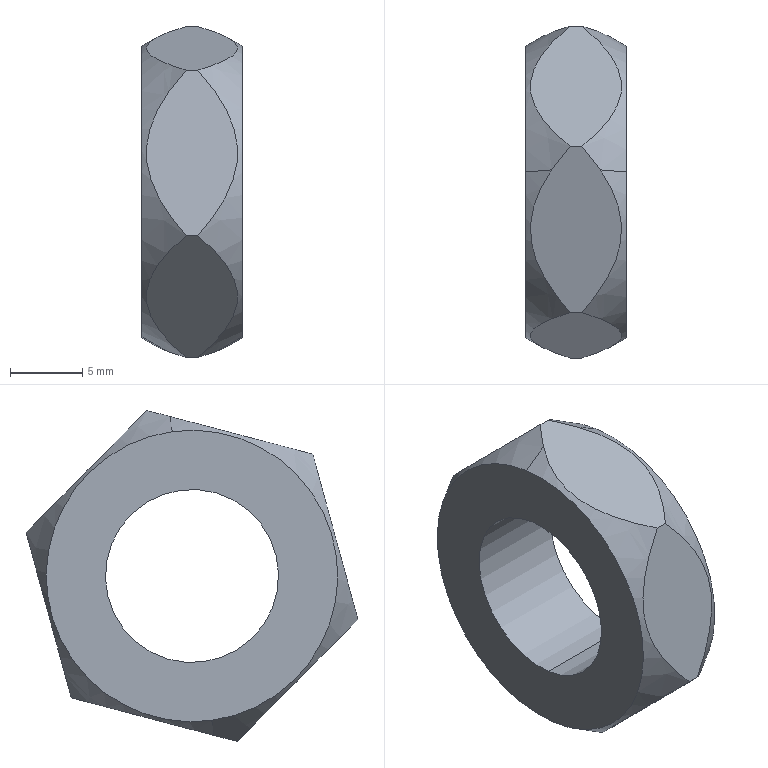Component | SolidWorks | NutM12-1 | 1 solid | 14 faces | box 7 x 23.01 x 22.95 mm | volume 1697 mm3 | plane 8 | cone 4 | cylinder 2 | commonest cylinder face diameters 12 x2
STEP:
#1=CARTESIAN_POINT('',(5.947,5.852,-0.9847));
#2=VERTEX_POINT('',#1);
#3=CARTESIAN_POINT('',(5.947,5.96,-0.1964));
#4=VERTEX_POINT('',#3);
#5=CARTESIAN_POINT('',(5.947,5.906,-0.5906));
#6=DIRECTION('',(1.,0.,0.));
#7=DIRECTION('',(0.,-0.1358,-0.9907));
#8=AXIS2_PLACEMENT_3D('',#5,#6,#7);
#9=CIRCLE('',#8,0.3978);
#10=EDGE_CURVE('',#2,#4,#9,.T.);
#11=ORIENTED_EDGE('',*,*,#10,.T.);
#12=CARTESIAN_POINT('',(6.018,5.965,-0.1556));
#13=VERTEX_POINT('',#12);
#14=CARTESIAN_POINT('',(5.947,5.96,-0.1964));
#15=DIRECTION('',(0.866,0.06788,0.4954));
#16=VECTOR('',#15,39.37);
#17=LINE('',#14,#16);
#18=EDGE_CURVE('',#4,#13,#17,.T.);
#19=ORIENTED_EDGE('',*,*,#18,.T.);
#20=CARTESIAN_POINT('',(6.069,6.029,-0.1388));
#21=VERTEX_POINT('',#20);
#22=CARTESIAN_POINT('',(6.069,6.029,-0.1388));
#23=CARTESIAN_POINT('',(6.051,6.008,-0.1442));
#24=CARTESIAN_POINT('',(6.034,5.987,-0.1497));
#25=CARTESIAN_POINT('',(6.018,5.965,-0.1556));
#26=B_SPLINE_CURVE_WITH_KNOTS('',3,(#22,#23,#24,#25),.UNSPECIFIED.,.F.,.F.,(4,4),(0.00000028,0.002105),.UNSPECIFIED.);
#27=EDGE_CURVE('',#21,#13,#26,.T.);
#28=ORIENTED_EDGE('',*,*,#27,.F.);
#29=CARTESIAN_POINT('',(6.069,6.358,-0.4715));
#30=VERTEX_POINT('',#29);
#31=CARTESIAN_POINT('',(6.069,6.358,-0.4715));
#32=CARTESIAN_POINT('',(6.054,6.347,-0.4597));
#33=CARTESIAN_POINT('',(6.041,6.335,-0.4475));
#34=CARTESIAN_POINT('',(6.015,6.31,-0.4222));
#35=CARTESIAN_POINT('',(6.004,6.297,-0.4091));
#36=CARTESIAN_POINT('',(5.984,6.269,-0.3814));
#37=CARTESIAN_POINT('',(5.975,6.255,-0.3667));
#38=CARTESIAN_POINT('',(5.966,6.232,-0.3442));
#39=CARTESIAN_POINT('',(5.964,6.225,-0.3366));
#40=CARTESIAN_POINT('',(5.961,6.209,-0.3211));
#41=CARTESIAN_POINT('',(5.96,6.202,-0.3131));
#42=CARTESIAN_POINT('',(5.96,6.178,-0.2897));
#43=CARTESIAN_POINT('',(5.963,6.163,-0.2743));
#44=CARTESIAN_POINT('',(5.975,6.133,-0.2439));
#45=CARTESIAN_POINT('',(5.983,6.119,-0.2295));
#46=CARTESIAN_POINT('',(6.003,6.091,-0.2018));
#47=CARTESIAN_POINT('',(6.015,6.078,-0.1885));
#48=CARTESIAN_POINT('',(6.041,6.053,-0.1629));
#49=CARTESIAN_POINT('',(6.054,6.041,-0.1507));
#50=CARTESIAN_POINT('',(6.069,6.029,-0.1388));
#51=B_SPLINE_CURVE_WITH_KNOTS('',3,(#31,#32,#33,#34,#35,#36,#37,#38,#39,#40,#41,#42,#43,#44,#45,#46,#47,#48,#49,#50),.UNSPECIFIED.,.F.,.F.,(4,2,2,2,2,2,2,2,2,4),(0.00000033,0.001663,0.003326,0.004989,0.005821,0.006652,0.008315,0.009978,0.01164,0.0133),.UNSPECIFIED.);
#52=EDGE_CURVE('',#30,#21,#51,.T.);
#53=ORIENTED_EDGE('',*,*,#52,.F.);
#54=CARTESIAN_POINT('',(6.069,6.235,-0.9232));
#55=VERTEX_POINT('',#54);
#56=CARTESIAN_POINT('',(6.069,6.235,-0.9232));
#57=CARTESIAN_POINT('',(6.054,6.239,-0.9072));
#58=CARTESIAN_POINT('',(6.041,6.244,-0.8907));
#59=CARTESIAN_POINT('',(6.015,6.253,-0.8563));
#60=CARTESIAN_POINT('',(6.004,6.258,-0.8385));
#61=CARTESIAN_POINT('',(5.984,6.268,-0.8009));
#62=CARTESIAN_POINT('',(5.975,6.274,-0.7809));
#63=CARTESIAN_POINT('',(5.966,6.282,-0.7504));
#64=CARTESIAN_POINT('',(5.964,6.285,-0.74));
#65=CARTESIAN_POINT('',(5.961,6.291,-0.7189));
#66=CARTESIAN_POINT('',(5.96,6.294,-0.7082));
#67=CARTESIAN_POINT('',(5.96,6.302,-0.6763));
#68=CARTESIAN_POINT('',(5.963,6.308,-0.6554));
#69=CARTESIAN_POINT('',(5.975,6.319,-0.6142));
#70=CARTESIAN_POINT('',(5.983,6.325,-0.5946));
#71=CARTESIAN_POINT('',(6.003,6.335,-0.557));
#72=CARTESIAN_POINT('',(6.015,6.34,-0.5389));
#73=CARTESIAN_POINT('',(6.041,6.349,-0.5042));
#74=CARTESIAN_POINT('',(6.054,6.354,-0.4876));
#75=CARTESIAN_POINT('',(6.069,6.358,-0.4715));
#76=B_SPLINE_CURVE_WITH_KNOTS('',3,(#56,#57,#58,#59,#60,#61,#62,#63,#64,#65,#66,#67,#68,#69,#70,#71,#72,#73,#74,#75),.UNSPECIFIED.,.F.,.F.,(4,2,2,2,2,2,2,2,2,4),(0.00000026,0.001663,0.003326,0.004989,0.00582,0.006652,0.008315,0.009978,0.01164,0.0133),.UNSPECIFIED.);
#77=EDGE_CURVE('',#55,#30,#76,.T.);
#78=ORIENTED_EDGE('',*,*,#77,.F.);
#79=CARTESIAN_POINT('',(6.018,5.846,-1.026));
#80=VERTEX_POINT('',#79);
#81=CARTESIAN_POINT('',(6.018,5.846,-1.026));
#82=CARTESIAN_POINT('',(6.008,5.861,-1.022));
#83=CARTESIAN_POINT('',(5.999,5.876,-1.018));
#84=CARTESIAN_POINT('',(5.982,5.908,-1.009));
#85=CARTESIAN_POINT('',(5.975,5.925,-1.005));
#86=CARTESIAN_POINT('',(5.968,5.951,-0.998));
#87=CARTESIAN_POINT('',(5.966,5.959,-0.9957));
#88=CARTESIAN_POINT('',(5.962,5.977,-0.991));
#89=CARTESIAN_POINT('',(5.961,5.986,-0.9887));
#90=CARTESIAN_POINT('',(5.96,6.013,-0.9816));
#91=CARTESIAN_POINT('',(5.961,6.031,-0.9769));
#92=CARTESIAN_POINT('',(5.967,6.066,-0.9677));
#93=CARTESIAN_POINT('',(5.972,6.084,-0.9631));
#94=CARTESIAN_POINT('',(5.986,6.117,-0.9543));
#95=CARTESIAN_POINT('',(5.994,6.133,-0.9501));
#96=CARTESIAN_POINT('',(6.013,6.164,-0.942));
#97=CARTESIAN_POINT('',(6.023,6.179,-0.9381));
#98=CARTESIAN_POINT('',(6.045,6.208,-0.9305));
#99=CARTESIAN_POINT('',(6.057,6.221,-0.9268));
#100=CARTESIAN_POINT('',(6.069,6.235,-0.9232));
#101=B_SPLINE_CURVE_WITH_KNOTS('',3,(#81,#82,#83,#84,#85,#86,#87,#88,#89,#90,#91,#92,#93,#94,#95,#96,#97,#98,#99,#100),.UNSPECIFIED.,.F.,.F.,(4,2,2,2,2,2,2,2,2,4),(0.002105,0.003505,0.004905,0.005605,0.006304,0.007704,0.009104,0.0105,0.0119,0.0133),.UNSPECIFIED.);
#102=EDGE_CURVE('',#80,#55,#101,.T.);
#103=ORIENTED_EDGE('',*,*,#102,.F.);
#104=CARTESIAN_POINT('',(5.947,5.852,-0.9847));
#105=DIRECTION('',(0.866,-0.06788,-0.4954));
#106=VECTOR('',#105,39.37);
#107=LINE('',#104,#106);
#108=EDGE_CURVE('',#2,#80,#107,.T.);
#109=ORIENTED_EDGE('',*,*,#108,.F.);
#110=EDGE_LOOP('',(#11,#19,#28,#53,#78,#103,#109));
#111=FACE_OUTER_BOUND('',#110,.T.);
#112=CARTESIAN_POINT('',(5.947,5.906,-0.5906));
#113=DIRECTION('',(1.,0.,0.));
#114=DIRECTION('',(0.,-0.1358,-0.9907));
#115=AXIS2_PLACEMENT_3D('',#112,#113,#114);
#116=CONICAL_SURFACE('',#115,0.3978,0.5236);
#117=ADVANCED_FACE('',(#111),#116,.T.);
#118=CARTESIAN_POINT('',(6.223,5.96,-0.1964));
#119=VERTEX_POINT('',#118);
#120=CARTESIAN_POINT('',(6.223,5.852,-0.9847));
#121=VERTEX_POINT('',#120);
#122=CARTESIAN_POINT('',(6.223,5.906,-0.5906));
#123=DIRECTION('',(1.,0.,0.));
#124=DIRECTION('',(0.,-0.1358,-0.9907));
#125=AXIS2_PLACEMENT_3D('',#122,#123,#124);
#126=CIRCLE('',#125,0.3978);
#127=EDGE_CURVE('',#119,#121,#126,.T.);
#128=ORIENTED_EDGE('',*,*,#127,.F.);
#129=CARTESIAN_POINT('',(6.151,5.965,-0.1556));
#130=VERTEX_POINT('',#129);
#131=CARTESIAN_POINT('',(6.223,5.96,-0.1964));
#132=DIRECTION('',(-0.866,0.06788,0.4954));
#133=VECTOR('',#132,39.37);
#134=LINE('',#131,#133);
#135=EDGE_CURVE('',#119,#130,#134,.T.);
#136=ORIENTED_EDGE('',*,*,#135,.T.);
#137=CARTESIAN_POINT('',(6.101,5.576,-0.2579));
#138=VERTEX_POINT('',#137);
#139=CARTESIAN_POINT('',(6.151,5.965,-0.1556));
#140=CARTESIAN_POINT('',(6.161,5.95,-0.1595));
#141=CARTESIAN_POINT('',(6.171,5.935,-0.1635));
#142=CARTESIAN_POINT('',(6.187,5.903,-0.1719));
#143=CARTESIAN_POINT('',(6.194,5.886,-0.1764));
#144=CARTESIAN_POINT('',(6.202,5.86,-0.1831));
#145=CARTESIAN_POINT('',(6.204,5.852,-0.1854));
#146=CARTESIAN_POINT('',(6.207,5.834,-0.1901));
#147=CARTESIAN_POINT('',(6.208,5.825,-0.1924));
#148=CARTESIAN_POINT('',(6.21,5.798,-0.1995));
#149=CARTESIAN_POINT('',(6.209,5.78,-0.2042));
#150=CARTESIAN_POINT('',(6.202,5.745,-0.2134));
#151=CARTESIAN_POINT('',(6.197,5.728,-0.218));
#152=CARTESIAN_POINT('',(6.184,5.694,-0.2268));
#153=CARTESIAN_POINT('',(6.175,5.678,-0.231));
#154=CARTESIAN_POINT('',(6.157,5.647,-0.2391));
#155=CARTESIAN_POINT('',(6.146,5.632,-0.243));
#156=CARTESIAN_POINT('',(6.124,5.604,-0.2506));
#157=CARTESIAN_POINT('',(6.113,5.59,-0.2543));
#158=CARTESIAN_POINT('',(6.101,5.576,-0.2579));
#159=B_SPLINE_CURVE_WITH_KNOTS('',3,(#139,#140,#141,#142,#143,#144,#145,#146,#147,#148,#149,#150,#151,#152,#153,#154,#155,#156,#157,#158),.UNSPECIFIED.,.F.,.F.,(4,2,2,2,2,2,2,2,2,4),(0.002105,0.003505,0.004905,0.005605,0.006304,0.007704,0.009104,0.0105,0.0119,0.0133),.UNSPECIFIED.);
#160=EDGE_CURVE('',#130,#138,#159,.T.);
#161=ORIENTED_EDGE('',*,*,#160,.T.);
#162=CARTESIAN_POINT('',(6.101,5.453,-0.7096));
#163=VERTEX_POINT('',#162);
#164=CARTESIAN_POINT('',(6.101,5.576,-0.2579));
#165=CARTESIAN_POINT('',(6.115,5.572,-0.2739));
#166=CARTESIAN_POINT('',(6.129,5.567,-0.2905));
#167=CARTESIAN_POINT('',(6.154,5.558,-0.3248));
#168=CARTESIAN_POINT('',(6.166,5.553,-0.3426));
#169=CARTESIAN_POINT('',(6.186,5.543,-0.3802));
#170=CARTESIAN_POINT('',(6.194,5.537,-0.4002));
#171=CARTESIAN_POINT('',(6.203,5.529,-0.4307));
#172=CARTESIAN_POINT('',(6.205,5.526,-0.4411));
#173=CARTESIAN_POINT('',(6.208,5.52,-0.4622));
#174=CARTESIAN_POINT('',(6.209,5.517,-0.4729));
#175=CARTESIAN_POINT('',(6.209,5.509,-0.5048));
#176=CARTESIAN_POINT('',(6.206,5.503,-0.5257));
#177=CARTESIAN_POINT('',(6.194,5.492,-0.5669));
#178=CARTESIAN_POINT('',(6.186,5.486,-0.5866));
#179=CARTESIAN_POINT('',(6.166,5.476,-0.6241));
#180=CARTESIAN_POINT('',(6.154,5.471,-0.6422));
#181=CARTESIAN_POINT('',(6.129,5.462,-0.6769));
#182=CARTESIAN_POINT('',(6.115,5.457,-0.6935));
#183=CARTESIAN_POINT('',(6.101,5.453,-0.7096));
#184=B_SPLINE_CURVE_WITH_KNOTS('',3,(#164,#165,#166,#167,#168,#169,#170,#171,#172,#173,#174,#175,#176,#177,#178,#179,#180,#181,#182,#183),.UNSPECIFIED.,.F.,.F.,(4,2,2,2,2,2,2,2,2,4),(0.00000026,0.001663,0.003326,0.004989,0.00582,0.006652,0.008315,0.009978,0.01164,0.0133),.UNSPECIFIED.);
#185=EDGE_CURVE('',#138,#163,#184,.T.);
#186=ORIENTED_EDGE('',*,*,#185,.T.);
#187=CARTESIAN_POINT('',(6.101,5.782,-1.042));
#188=VERTEX_POINT('',#187);
#189=CARTESIAN_POINT('',(6.101,5.453,-0.7096));
#190=CARTESIAN_POINT('',(6.115,5.464,-0.7214));
#191=CARTESIAN_POINT('',(6.129,5.476,-0.7336));
#192=CARTESIAN_POINT('',(6.154,5.501,-0.7589));
#193=CARTESIAN_POINT('',(6.166,5.514,-0.772));
#194=CARTESIAN_POINT('',(6.186,5.542,-0.7997));
#195=CARTESIAN_POINT('',(6.194,5.556,-0.8144));
#196=CARTESIAN_POINT('',(6.203,5.579,-0.8369));
#197=CARTESIAN_POINT('',(6.205,5.586,-0.8445));
#198=CARTESIAN_POINT('',(6.208,5.602,-0.8601));
#199=CARTESIAN_POINT('',(6.209,5.61,-0.868));
#200=CARTESIAN_POINT('',(6.209,5.633,-0.8914));
#201=CARTESIAN_POINT('',(6.206,5.648,-0.9068));
#202=CARTESIAN_POINT('',(6.194,5.678,-0.9372));
#203=CARTESIAN_POINT('',(6.186,5.692,-0.9517));
#204=CARTESIAN_POINT('',(6.166,5.72,-0.9793));
#205=CARTESIAN_POINT('',(6.154,5.733,-0.9926));
#206=CARTESIAN_POINT('',(6.129,5.758,-1.018));
#207=CARTESIAN_POINT('',(6.115,5.77,-1.03));
#208=CARTESIAN_POINT('',(6.101,5.782,-1.042));
#209=B_SPLINE_CURVE_WITH_KNOTS('',3,(#189,#190,#191,#192,#193,#194,#195,#196,#197,#198,#199,#200,#201,#202,#203,#204,#205,#206,#207,#208),.UNSPECIFIED.,.F.,.F.,(4,2,2,2,2,2,2,2,2,4),(0.00000033,0.001663,0.003326,0.004989,0.005821,0.006652,0.008315,0.009978,0.01164,0.0133),.UNSPECIFIED.);
#210=EDGE_CURVE('',#163,#188,#209,.T.);
#211=ORIENTED_EDGE('',*,*,#210,.T.);
#212=CARTESIAN_POINT('',(6.151,5.846,-1.026));
#213=VERTEX_POINT('',#212);
#214=CARTESIAN_POINT('',(6.101,5.782,-1.042));
#215=CARTESIAN_POINT('',(6.119,5.803,-1.037));
#216=CARTESIAN_POINT('',(6.136,5.824,-1.031));
#217=CARTESIAN_POINT('',(6.151,5.846,-1.026));
#218=B_SPLINE_CURVE_WITH_KNOTS('',3,(#214,#215,#216,#217),.UNSPECIFIED.,.F.,.F.,(4,4),(0.00000028,0.002105),.UNSPECIFIED.);
#219=EDGE_CURVE('',#188,#213,#218,.T.);
#220=ORIENTED_EDGE('',*,*,#219,.T.);
#221=CARTESIAN_POINT('',(6.223,5.852,-0.9847));
#222=DIRECTION('',(-0.866,-0.06788,-0.4954));
#223=VECTOR('',#222,39.37);
#224=LINE('',#221,#223);
#225=EDGE_CURVE('',#121,#213,#224,.T.);
#226=ORIENTED_EDGE('',*,*,#225,.F.);
#227=EDGE_LOOP('',(#128,#136,#161,#186,#211,#220,#226));
#228=FACE_OUTER_BOUND('',#227,.T.);
#229=CARTESIAN_POINT('',(6.223,5.906,-0.5906));
#230=DIRECTION('',(-1.,0.,0.));
#231=DIRECTION('',(0.,-0.1358,-0.9907));
#232=AXIS2_PLACEMENT_3D('',#229,#230,#231);
#233=CONICAL_SURFACE('',#232,0.3978,0.5236);
#234=ADVANCED_FACE('',(#228),#233,.T.);
#235=CARTESIAN_POINT('',(6.223,5.938,-0.3565));
#236=VERTEX_POINT('',#235);
#237=CARTESIAN_POINT('',(6.223,5.873,-0.8246));
#238=VERTEX_POINT('',#237);
#239=CARTESIAN_POINT('',(6.223,5.906,-0.5906));
#240=DIRECTION('',(1.,0.,0.));
#241=DIRECTION('',(0.,-0.1358,-0.9907));
#242=AXIS2_PLACEMENT_3D('',#239,#240,#241);
#243=CIRCLE('',#242,0.2362);
#244=EDGE_CURVE('',#236,#238,#243,.T.);
#245=ORIENTED_EDGE('',*,*,#244,.T.);
#246=CARTESIAN_POINT('',(5.947,5.873,-0.8246));
#247=VERTEX_POINT('',#246);
#248=CARTESIAN_POINT('',(6.223,5.873,-0.8246));
#249=DIRECTION('',(-1.,0.,0.));
#250=VECTOR('',#249,39.37);
#251=LINE('',#248,#250);
#252=EDGE_CURVE('',#238,#247,#251,.T.);
#253=ORIENTED_EDGE('',*,*,#252,.T.);
#254=CARTESIAN_POINT('',(5.947,5.938,-0.3565));
#255=VERTEX_POINT('',#254);
#256=CARTESIAN_POINT('',(5.947,5.906,-0.5906));
#257=DIRECTION('',(1.,0.,0.));
#258=DIRECTION('',(0.,-0.1358,-0.9907));
#259=AXIS2_PLACEMENT_3D('',#256,#257,#258);
#260=CIRCLE('',#259,0.2362);
#261=EDGE_CURVE('',#255,#247,#260,.T.);
#262=ORIENTED_EDGE('',*,*,#261,.F.);
#263=CARTESIAN_POINT('',(6.223,5.938,-0.3565));
#264=DIRECTION('',(-1.,0.,0.));
#265=VECTOR('',#264,39.37);
#266=LINE('',#263,#265);
#267=EDGE_CURVE('',#236,#255,#266,.T.);
#268=ORIENTED_EDGE('',*,*,#267,.F.);
#269=EDGE_LOOP('',(#245,#253,#262,#268));
#270=FACE_OUTER_BOUND('',#269,.T.);
#271=CARTESIAN_POINT('',(6.223,5.906,-0.5906));
#272=DIRECTION('',(-1.,0.,0.));
#273=DIRECTION('',(0.,0.1358,0.9907));
#274=AXIS2_PLACEMENT_3D('',#271,#272,#273);
#275=CYLINDRICAL_SURFACE('',#274,0.2362);
#276=ADVANCED_FACE('',(#270),#275,.F.);
#277=ORIENTED_EDGE('',*,*,#261,.T.);
#278=CARTESIAN_POINT('',(5.947,5.906,-0.5906));
#279=DIRECTION('',(1.,0.,0.));
#280=DIRECTION('',(0.,-0.1358,-0.9907));
#281=AXIS2_PLACEMENT_3D('',#278,#279,#280);
#282=CIRCLE('',#281,0.2362);
#283=EDGE_CURVE('',#247,#255,#282,.T.);
#284=ORIENTED_EDGE('',*,*,#283,.T.);
#285=EDGE_LOOP('',(#277,#284));
#286=FACE_BOUND('',#285,.T.);
#287=ORIENTED_EDGE('',*,*,#10,.F.);
#288=CARTESIAN_POINT('',(5.947,5.906,-0.5906));
#289=DIRECTION('',(1.,0.,0.));
#290=DIRECTION('',(0.,-0.1358,-0.9907));
#291=AXIS2_PLACEMENT_3D('',#288,#289,#290);
#292=CIRCLE('',#291,0.3978);
#293=EDGE_CURVE('',#4,#2,#292,.T.);
#294=ORIENTED_EDGE('',*,*,#293,.F.);
#295=EDGE_LOOP('',(#287,#294));
#296=FACE_OUTER_BOUND('',#295,.T.);
#297=CARTESIAN_POINT('',(5.947,0.1348,0.7962));
#298=DIRECTION('',(1.,0.,0.));
#299=DIRECTION('',(0.,-0.1358,-0.9907));
#300=AXIS2_PLACEMENT_3D('',#297,#298,#299);
#301=PLANE('',#300);
#302=ADVANCED_FACE('',(#286,#296),#301,.F.);
#303=ORIENTED_EDGE('',*,*,#244,.F.);
#304=CARTESIAN_POINT('',(6.223,5.906,-0.5906));
#305=DIRECTION('',(1.,0.,0.));
#306=DIRECTION('',(0.,-0.1358,-0.9907));
#307=AXIS2_PLACEMENT_3D('',#304,#305,#306);
#308=CIRCLE('',#307,0.2362);
#309=EDGE_CURVE('',#238,#236,#308,.T.);
#310=ORIENTED_EDGE('',*,*,#309,.F.);
#311=EDGE_LOOP('',(#303,#310));
#312=FACE_BOUND('',#311,.T.);
#313=CARTESIAN_POINT('',(6.223,5.906,-0.5906));
#314=DIRECTION('',(1.,0.,0.));
#315=DIRECTION('',(0.,-0.1358,-0.9907));
#316=AXIS2_PLACEMENT_3D('',#313,#314,#315);
#317=CIRCLE('',#316,0.3978);
#318=EDGE_CURVE('',#121,#119,#317,.T.);
#319=ORIENTED_EDGE('',*,*,#318,.T.);
#320=ORIENTED_EDGE('',*,*,#127,.T.);
#321=EDGE_LOOP('',(#319,#320));
#322=FACE_OUTER_BOUND('',#321,.T.);
#323=CARTESIAN_POINT('',(6.223,0.1348,0.7962));
#324=DIRECTION('',(1.,0.,0.));
#325=DIRECTION('',(0.,-0.1358,-0.9907));
#326=AXIS2_PLACEMENT_3D('',#323,#324,#325);
#327=PLANE('',#326);
#328=ADVANCED_FACE('',(#312,#322),#327,.T.);
#329=CARTESIAN_POINT('',(6.069,5.782,-1.042));
#330=VERTEX_POINT('',#329);
#331=CARTESIAN_POINT('',(6.223,5.782,-1.042));
#332=DIRECTION('',(-1.,0.,0.));
#333=VECTOR('',#332,39.37);
#334=LINE('',#331,#333);
#335=EDGE_CURVE('',#188,#330,#334,.T.);
#336=ORIENTED_EDGE('',*,*,#335,.T.);
#337=CARTESIAN_POINT('',(6.069,5.782,-1.042));
#338=CARTESIAN_POINT('',(6.051,5.803,-1.037));
#339=CARTESIAN_POINT('',(6.034,5.824,-1.031));
#340=CARTESIAN_POINT('',(6.018,5.846,-1.026));
#341=B_SPLINE_CURVE_WITH_KNOTS('',3,(#337,#338,#339,#340),.UNSPECIFIED.,.F.,.F.,(4,4),(0.00000028,0.002105),.UNSPECIFIED.);
#342=EDGE_CURVE('',#330,#80,#341,.T.);
#343=ORIENTED_EDGE('',*,*,#342,.T.);
#344=ORIENTED_EDGE('',*,*,#102,.T.);
#345=CARTESIAN_POINT('',(6.101,6.235,-0.9232));
#346=VERTEX_POINT('',#345);
#347=CARTESIAN_POINT('',(6.223,6.235,-0.9232));
#348=DIRECTION('',(-1.,0.,0.));
#349=VECTOR('',#348,39.37);
#350=LINE('',#347,#349);
#351=EDGE_CURVE('',#346,#55,#350,.T.);
#352=ORIENTED_EDGE('',*,*,#351,.F.);
#353=CARTESIAN_POINT('',(6.151,5.846,-1.026));
#354=CARTESIAN_POINT('',(6.161,5.861,-1.022));
#355=CARTESIAN_POINT('',(6.171,5.876,-1.018));
#356=CARTESIAN_POINT('',(6.187,5.908,-1.009));
#357=CARTESIAN_POINT('',(6.194,5.925,-1.005));
#358=CARTESIAN_POINT('',(6.202,5.951,-0.998));
#359=CARTESIAN_POINT('',(6.204,5.959,-0.9957));
#360=CARTESIAN_POINT('',(6.207,5.977,-0.991));
#361=CARTESIAN_POINT('',(6.208,5.986,-0.9887));
#362=CARTESIAN_POINT('',(6.21,6.013,-0.9816));
#363=CARTESIAN_POINT('',(6.209,6.031,-0.9769));
#364=CARTESIAN_POINT('',(6.202,6.066,-0.9677));
#365=CARTESIAN_POINT('',(6.197,6.084,-0.9631));
#366=CARTESIAN_POINT('',(6.184,6.117,-0.9543));
#367=CARTESIAN_POINT('',(6.175,6.133,-0.9501));
#368=CARTESIAN_POINT('',(6.157,6.164,-0.942));
#369=CARTESIAN_POINT('',(6.146,6.179,-0.9381));
#370=CARTESIAN_POINT('',(6.124,6.208,-0.9305));
#371=CARTESIAN_POINT('',(6.113,6.221,-0.9268));
#372=CARTESIAN_POINT('',(6.101,6.235,-0.9232));
#373=B_SPLINE_CURVE_WITH_KNOTS('',3,(#353,#354,#355,#356,#357,#358,#359,#360,#361,#362,#363,#364,#365,#366,#367,#368,#369,#370,#371,#372),.UNSPECIFIED.,.F.,.F.,(4,2,2,2,2,2,2,2,2,4),(0.002105,0.003505,0.004905,0.005605,0.006304,0.007704,0.009104,0.0105,0.0119,0.0133),.UNSPECIFIED.);
#374=EDGE_CURVE('',#213,#346,#373,.T.);
#375=ORIENTED_EDGE('',*,*,#374,.F.);
#376=ORIENTED_EDGE('',*,*,#219,.F.);
#377=EDGE_LOOP('',(#336,#343,#344,#352,#375,#376));
#378=FACE_OUTER_BOUND('',#377,.T.);
#379=CARTESIAN_POINT('',(6.223,5.782,-1.042));
#380=DIRECTION('',(0.,-0.2543,0.9671));
#381=DIRECTION('',(0.,-0.9671,-0.2543));
#382=AXIS2_PLACEMENT_3D('',#379,#380,#381);
#383=PLANE('',#382);
#384=ADVANCED_FACE('',(#378),#383,.F.);
#385=ORIENTED_EDGE('',*,*,#351,.T.);
#386=ORIENTED_EDGE('',*,*,#77,.T.);
#387=CARTESIAN_POINT('',(6.101,6.358,-0.4715));
#388=VERTEX_POINT('',#387);
#389=CARTESIAN_POINT('',(6.223,6.358,-0.4715));
#390=DIRECTION('',(-1.,0.,0.));
#391=VECTOR('',#390,39.37);
#392=LINE('',#389,#391);
#393=EDGE_CURVE('',#388,#30,#392,.T.);
#394=ORIENTED_EDGE('',*,*,#393,.F.);
#395=CARTESIAN_POINT('',(6.101,6.235,-0.9232));
#396=CARTESIAN_POINT('',(6.115,6.239,-0.9072));
#397=CARTESIAN_POINT('',(6.129,6.244,-0.8907));
#398=CARTESIAN_POINT('',(6.154,6.253,-0.8563));
#399=CARTESIAN_POINT('',(6.166,6.258,-0.8385));
#400=CARTESIAN_POINT('',(6.186,6.268,-0.8009));
#401=CARTESIAN_POINT('',(6.194,6.274,-0.7809));
#402=CARTESIAN_POINT('',(6.203,6.282,-0.7504));
#403=CARTESIAN_POINT('',(6.205,6.285,-0.74));
#404=CARTESIAN_POINT('',(6.208,6.291,-0.7189));
#405=CARTESIAN_POINT('',(6.209,6.294,-0.7082));
#406=CARTESIAN_POINT('',(6.209,6.302,-0.6763));
#407=CARTESIAN_POINT('',(6.206,6.308,-0.6554));
#408=CARTESIAN_POINT('',(6.194,6.319,-0.6142));
#409=CARTESIAN_POINT('',(6.186,6.325,-0.5946));
#410=CARTESIAN_POINT('',(6.166,6.335,-0.557));
#411=CARTESIAN_POINT('',(6.154,6.34,-0.5389));
#412=CARTESIAN_POINT('',(6.129,6.349,-0.5042));
#413=CARTESIAN_POINT('',(6.115,6.354,-0.4876));
#414=CARTESIAN_POINT('',(6.101,6.358,-0.4715));
#415=B_SPLINE_CURVE_WITH_KNOTS('',3,(#395,#396,#397,#398,#399,#400,#401,#402,#403,#404,#405,#406,#407,#408,#409,#410,#411,#412,#413,#414),.UNSPECIFIED.,.F.,.F.,(4,2,2,2,2,2,2,2,2,4),(0.00000026,0.001663,0.003326,0.004989,0.00582,0.006652,0.008315,0.009978,0.01164,0.0133),.UNSPECIFIED.);
#416=EDGE_CURVE('',#346,#388,#415,.T.);
#417=ORIENTED_EDGE('',*,*,#416,.F.);
#418=EDGE_LOOP('',(#385,#386,#394,#417));
#419=FACE_OUTER_BOUND('',#418,.T.);
#420=CARTESIAN_POINT('',(6.223,6.235,-0.9232));
#421=DIRECTION('',(0.,-0.9647,0.2634));
#422=DIRECTION('',(0.,-0.2634,-0.9647));
#423=AXIS2_PLACEMENT_3D('',#420,#421,#422);
#424=PLANE('',#423);
#425=ADVANCED_FACE('',(#419),#424,.F.);
#426=ORIENTED_EDGE('',*,*,#393,.T.);
#427=ORIENTED_EDGE('',*,*,#52,.T.);
#428=CARTESIAN_POINT('',(6.101,6.029,-0.1388));
#429=VERTEX_POINT('',#428);
#430=CARTESIAN_POINT('',(6.223,6.029,-0.1388));
#431=DIRECTION('',(-1.,0.,0.));
#432=VECTOR('',#431,39.37);
#433=LINE('',#430,#432);
#434=EDGE_CURVE('',#429,#21,#433,.T.);
#435=ORIENTED_EDGE('',*,*,#434,.F.);
#436=CARTESIAN_POINT('',(6.101,6.358,-0.4715));
#437=CARTESIAN_POINT('',(6.115,6.347,-0.4597));
#438=CARTESIAN_POINT('',(6.129,6.335,-0.4475));
#439=CARTESIAN_POINT('',(6.154,6.31,-0.4222));
#440=CARTESIAN_POINT('',(6.166,6.297,-0.4091));
#441=CARTESIAN_POINT('',(6.186,6.269,-0.3814));
#442=CARTESIAN_POINT('',(6.194,6.255,-0.3667));
#443=CARTESIAN_POINT('',(6.203,6.232,-0.3442));
#444=CARTESIAN_POINT('',(6.205,6.225,-0.3366));
#445=CARTESIAN_POINT('',(6.208,6.209,-0.3211));
#446=CARTESIAN_POINT('',(6.209,6.202,-0.3131));
#447=CARTESIAN_POINT('',(6.209,6.178,-0.2897));
#448=CARTESIAN_POINT('',(6.206,6.163,-0.2743));
#449=CARTESIAN_POINT('',(6.194,6.133,-0.2439));
#450=CARTESIAN_POINT('',(6.186,6.119,-0.2295));
#451=CARTESIAN_POINT('',(6.166,6.091,-0.2018));
#452=CARTESIAN_POINT('',(6.154,6.078,-0.1885));
#453=CARTESIAN_POINT('',(6.129,6.053,-0.1629));
#454=CARTESIAN_POINT('',(6.115,6.041,-0.1507));
#455=CARTESIAN_POINT('',(6.101,6.029,-0.1388));
#456=B_SPLINE_CURVE_WITH_KNOTS('',3,(#436,#437,#438,#439,#440,#441,#442,#443,#444,#445,#446,#447,#448,#449,#450,#451,#452,#453,#454,#455),.UNSPECIFIED.,.F.,.F.,(4,2,2,2,2,2,2,2,2,4),(0.00000033,0.001663,0.003326,0.004989,0.005821,0.006652,0.008315,0.009978,0.01164,0.0133),.UNSPECIFIED.);
#457=EDGE_CURVE('',#388,#429,#456,.T.);
#458=ORIENTED_EDGE('',*,*,#457,.F.);
#459=EDGE_LOOP('',(#426,#427,#435,#458));
#460=FACE_OUTER_BOUND('',#459,.T.);
#461=CARTESIAN_POINT('',(6.223,6.358,-0.4715));
#462=DIRECTION('',(0.,-0.7104,-0.7038));
#463=DIRECTION('',(0.,0.7038,-0.7104));
#464=AXIS2_PLACEMENT_3D('',#461,#462,#463);
#465=PLANE('',#464);
#466=ADVANCED_FACE('',(#460),#465,.F.);
#467=ORIENTED_EDGE('',*,*,#434,.T.);
#468=ORIENTED_EDGE('',*,*,#27,.T.);
#469=CARTESIAN_POINT('',(6.069,5.576,-0.2579));
#470=VERTEX_POINT('',#469);
#471=CARTESIAN_POINT('',(6.018,5.965,-0.1556));
#472=CARTESIAN_POINT('',(6.008,5.95,-0.1595));
#473=CARTESIAN_POINT('',(5.999,5.935,-0.1635));
#474=CARTESIAN_POINT('',(5.982,5.903,-0.1719));
#475=CARTESIAN_POINT('',(5.975,5.886,-0.1764));
#476=CARTESIAN_POINT('',(5.968,5.86,-0.1831));
#477=CARTESIAN_POINT('',(5.966,5.852,-0.1854));
#478=CARTESIAN_POINT('',(5.962,5.834,-0.1901));
#479=CARTESIAN_POINT('',(5.961,5.825,-0.1924));
#480=CARTESIAN_POINT('',(5.96,5.798,-0.1995));
#481=CARTESIAN_POINT('',(5.961,5.78,-0.2042));
#482=CARTESIAN_POINT('',(5.967,5.745,-0.2134));
#483=CARTESIAN_POINT('',(5.972,5.728,-0.218));
#484=CARTESIAN_POINT('',(5.986,5.694,-0.2268));
#485=CARTESIAN_POINT('',(5.994,5.678,-0.231));
#486=CARTESIAN_POINT('',(6.013,5.647,-0.2391));
#487=CARTESIAN_POINT('',(6.023,5.632,-0.243));
#488=CARTESIAN_POINT('',(6.045,5.604,-0.2506));
#489=CARTESIAN_POINT('',(6.057,5.59,-0.2543));
#490=CARTESIAN_POINT('',(6.069,5.576,-0.2579));
#491=B_SPLINE_CURVE_WITH_KNOTS('',3,(#471,#472,#473,#474,#475,#476,#477,#478,#479,#480,#481,#482,#483,#484,#485,#486,#487,#488,#489,#490),.UNSPECIFIED.,.F.,.F.,(4,2,2,2,2,2,2,2,2,4),(0.002105,0.003505,0.004905,0.005605,0.006304,0.007704,0.009104,0.0105,0.0119,0.0133),.UNSPECIFIED.);
#492=EDGE_CURVE('',#13,#470,#491,.T.);
#493=ORIENTED_EDGE('',*,*,#492,.T.);
#494=CARTESIAN_POINT('',(6.223,5.576,-0.2579));
#495=DIRECTION('',(-1.,0.,0.));
#496=VECTOR('',#495,39.37);
#497=LINE('',#494,#496);
#498=EDGE_CURVE('',#138,#470,#497,.T.);
#499=ORIENTED_EDGE('',*,*,#498,.F.);
#500=ORIENTED_EDGE('',*,*,#160,.F.);
#501=CARTESIAN_POINT('',(6.101,6.029,-0.1388));
#502=CARTESIAN_POINT('',(6.119,6.008,-0.1442));
#503=CARTESIAN_POINT('',(6.136,5.987,-0.1497));
#504=CARTESIAN_POINT('',(6.151,5.965,-0.1556));
#505=B_SPLINE_CURVE_WITH_KNOTS('',3,(#501,#502,#503,#504),.UNSPECIFIED.,.F.,.F.,(4,4),(0.00000028,0.002105),.UNSPECIFIED.);
#506=EDGE_CURVE('',#429,#130,#505,.T.);
#507=ORIENTED_EDGE('',*,*,#506,.F.);
#508=EDGE_LOOP('',(#467,#468,#493,#499,#500,#507));
#509=FACE_OUTER_BOUND('',#508,.T.);
#510=CARTESIAN_POINT('',(6.223,6.029,-0.1388));
#511=DIRECTION('',(0.,0.2543,-0.9671));
#512=DIRECTION('',(0.,0.9671,0.2543));
#513=AXIS2_PLACEMENT_3D('',#510,#511,#512);
#514=PLANE('',#513);
#515=ADVANCED_FACE('',(#509),#514,.F.);
#516=ORIENTED_EDGE('',*,*,#498,.T.);
#517=CARTESIAN_POINT('',(6.069,5.453,-0.7096));
#518=VERTEX_POINT('',#517);
#519=CARTESIAN_POINT('',(6.069,5.576,-0.2579));
#520=CARTESIAN_POINT('',(6.054,5.572,-0.2739));
#521=CARTESIAN_POINT('',(6.041,5.567,-0.2905));
#522=CARTESIAN_POINT('',(6.015,5.558,-0.3248));
#523=CARTESIAN_POINT('',(6.004,5.553,-0.3426));
#524=CARTESIAN_POINT('',(5.984,5.543,-0.3802));
#525=CARTESIAN_POINT('',(5.975,5.537,-0.4002));
#526=CARTESIAN_POINT('',(5.966,5.529,-0.4307));
#527=CARTESIAN_POINT('',(5.964,5.526,-0.4411));
#528=CARTESIAN_POINT('',(5.961,5.52,-0.4622));
#529=CARTESIAN_POINT('',(5.96,5.517,-0.4729));
#530=CARTESIAN_POINT('',(5.96,5.509,-0.5048));
#531=CARTESIAN_POINT('',(5.963,5.503,-0.5257));
#532=CARTESIAN_POINT('',(5.975,5.492,-0.5669));
#533=CARTESIAN_POINT('',(5.983,5.486,-0.5866));
#534=CARTESIAN_POINT('',(6.003,5.476,-0.6241));
#535=CARTESIAN_POINT('',(6.015,5.471,-0.6422));
#536=CARTESIAN_POINT('',(6.041,5.462,-0.6769));
#537=CARTESIAN_POINT('',(6.054,5.457,-0.6935));
#538=CARTESIAN_POINT('',(6.069,5.453,-0.7096));
#539=B_SPLINE_CURVE_WITH_KNOTS('',3,(#519,#520,#521,#522,#523,#524,#525,#526,#527,#528,#529,#530,#531,#532,#533,#534,#535,#536,#537,#538),.UNSPECIFIED.,.F.,.F.,(4,2,2,2,2,2,2,2,2,4),(0.00000026,0.001663,0.003326,0.004989,0.00582,0.006652,0.008315,0.009978,0.01164,0.0133),.UNSPECIFIED.);
#540=EDGE_CURVE('',#470,#518,#539,.T.);
#541=ORIENTED_EDGE('',*,*,#540,.T.);
#542=CARTESIAN_POINT('',(6.223,5.453,-0.7096));
#543=DIRECTION('',(-1.,0.,0.));
#544=VECTOR('',#543,39.37);
#545=LINE('',#542,#544);
#546=EDGE_CURVE('',#163,#518,#545,.T.);
#547=ORIENTED_EDGE('',*,*,#546,.F.);
#548=ORIENTED_EDGE('',*,*,#185,.F.);
#549=EDGE_LOOP('',(#516,#541,#547,#548));
#550=FACE_OUTER_BOUND('',#549,.T.);
#551=CARTESIAN_POINT('',(6.223,5.576,-0.2579));
#552=DIRECTION('',(0.,0.9647,-0.2634));
#553=DIRECTION('',(0.,0.2634,0.9647));
#554=AXIS2_PLACEMENT_3D('',#551,#552,#553);
#555=PLANE('',#554);
#556=ADVANCED_FACE('',(#550),#555,.F.);
#557=ORIENTED_EDGE('',*,*,#546,.T.);
#558=CARTESIAN_POINT('',(6.069,5.453,-0.7096));
#559=CARTESIAN_POINT('',(6.054,5.464,-0.7214));
#560=CARTESIAN_POINT('',(6.041,5.476,-0.7336));
#561=CARTESIAN_POINT('',(6.015,5.501,-0.7589));
#562=CARTESIAN_POINT('',(6.004,5.514,-0.772));
#563=CARTESIAN_POINT('',(5.984,5.542,-0.7997));
#564=CARTESIAN_POINT('',(5.975,5.556,-0.8144));
#565=CARTESIAN_POINT('',(5.966,5.579,-0.8369));
#566=CARTESIAN_POINT('',(5.964,5.586,-0.8445));
#567=CARTESIAN_POINT('',(5.961,5.602,-0.8601));
#568=CARTESIAN_POINT('',(5.96,5.61,-0.868));
#569=CARTESIAN_POINT('',(5.96,5.633,-0.8914));
#570=CARTESIAN_POINT('',(5.963,5.648,-0.9068));
#571=CARTESIAN_POINT('',(5.975,5.678,-0.9372));
#572=CARTESIAN_POINT('',(5.983,5.692,-0.9517));
#573=CARTESIAN_POINT('',(6.003,5.72,-0.9793));
#574=CARTESIAN_POINT('',(6.015,5.733,-0.9926));
#575=CARTESIAN_POINT('',(6.041,5.758,-1.018));
#576=CARTESIAN_POINT('',(6.054,5.77,-1.03));
#577=CARTESIAN_POINT('',(6.069,5.782,-1.042));
#578=B_SPLINE_CURVE_WITH_KNOTS('',3,(#558,#559,#560,#561,#562,#563,#564,#565,#566,#567,#568,#569,#570,#571,#572,#573,#574,#575,#576,#577),.UNSPECIFIED.,.F.,.F.,(4,2,2,2,2,2,2,2,2,4),(0.00000033,0.001663,0.003326,0.004989,0.005821,0.006652,0.008315,0.009978,0.01164,0.0133),.UNSPECIFIED.);
#579=EDGE_CURVE('',#518,#330,#578,.T.);
#580=ORIENTED_EDGE('',*,*,#579,.T.);
#581=ORIENTED_EDGE('',*,*,#335,.F.);
#582=ORIENTED_EDGE('',*,*,#210,.F.);
#583=EDGE_LOOP('',(#557,#580,#581,#582));
#584=FACE_OUTER_BOUND('',#583,.T.);
#585=CARTESIAN_POINT('',(6.223,5.453,-0.7096));
#586=DIRECTION('',(0.,0.7104,0.7038));
#587=DIRECTION('',(0.,-0.7038,0.7104));
#588=AXIS2_PLACEMENT_3D('',#585,#586,#587);
#589=PLANE('',#588);
#590=ADVANCED_FACE('',(#584),#589,.F.);
#591=ORIENTED_EDGE('',*,*,#252,.F.);
#592=ORIENTED_EDGE('',*,*,#309,.T.);
#593=ORIENTED_EDGE('',*,*,#267,.T.);
#594=ORIENTED_EDGE('',*,*,#283,.F.);
#595=EDGE_LOOP('',(#591,#592,#593,#594));
#596=FACE_OUTER_BOUND('',#595,.T.);
#597=CARTESIAN_POINT('',(6.223,5.906,-0.5906));
#598=DIRECTION('',(-1.,0.,0.));
#599=DIRECTION('',(0.,0.1358,0.9907));
#600=AXIS2_PLACEMENT_3D('',#597,#598,#599);
#601=CYLINDRICAL_SURFACE('',#600,0.2362);
#602=ADVANCED_FACE('',(#596),#601,.F.);
#603=ORIENTED_EDGE('',*,*,#135,.F.);
#604=ORIENTED_EDGE('',*,*,#318,.F.);
#605=ORIENTED_EDGE('',*,*,#225,.T.);
#606=ORIENTED_EDGE('',*,*,#374,.T.);
#607=ORIENTED_EDGE('',*,*,#416,.T.);
#608=ORIENTED_EDGE('',*,*,#457,.T.);
#609=ORIENTED_EDGE('',*,*,#506,.T.);
#610=EDGE_LOOP('',(#603,#604,#605,#606,#607,#608,#609));
#611=FACE_OUTER_BOUND('',#610,.T.);
#612=CARTESIAN_POINT('',(6.223,5.906,-0.5906));
#613=DIRECTION('',(-1.,0.,0.));
#614=DIRECTION('',(0.,-0.1358,-0.9907));
#615=AXIS2_PLACEMENT_3D('',#612,#613,#614);
#616=CONICAL_SURFACE('',#615,0.3978,0.5236);
#617=ADVANCED_FACE('',(#611),#616,.T.);
#618=ORIENTED_EDGE('',*,*,#18,.F.);
#619=ORIENTED_EDGE('',*,*,#293,.T.);
#620=ORIENTED_EDGE('',*,*,#108,.T.);
#621=ORIENTED_EDGE('',*,*,#342,.F.);
#622=ORIENTED_EDGE('',*,*,#579,.F.);
#623=ORIENTED_EDGE('',*,*,#540,.F.);
#624=ORIENTED_EDGE('',*,*,#492,.F.);
#625=EDGE_LOOP('',(#618,#619,#620,#621,#622,#623,#624));
#626=FACE_OUTER_BOUND('',#625,.T.);
#627=CARTESIAN_POINT('',(5.947,5.906,-0.5906));
#628=DIRECTION('',(1.,0.,0.));
#629=DIRECTION('',(0.,-0.1358,-0.9907));
#630=AXIS2_PLACEMENT_3D('',#627,#628,#629);
#631=CONICAL_SURFACE('',#630,0.3978,0.5236);
#632=ADVANCED_FACE('',(#626),#631,.T.);
#633=CLOSED_SHELL('',(#117,#234,#276,#302,#328,#384,#425,#466,#515,#556,#590,#602,#617,#632));
#634=MANIFOLD_SOLID_BREP('',#633);
#635=CARTESIAN_POINT('',(0.,0.,0.));
#636=DIRECTION('',(0.,0.,1.));
#637=DIRECTION('',(1.,0.,0.));
#638=AXIS2_PLACEMENT_3D('',#635,#636,#637);
#639=(LENGTH_UNIT()NAMED_UNIT(*)SI_UNIT($,.METRE.));
#640=LENGTH_MEASURE_WITH_UNIT(LENGTH_MEASURE(0.0254),#639);
#641=DIMENSIONAL_EXPONENTS(1.,0.,0.,0.,0.,0.,0.);
#642=(CONVERSION_BASED_UNIT('',#640)LENGTH_UNIT()NAMED_UNIT(#641));
#643=UNCERTAINTY_MEASURE_WITH_UNIT(LENGTH_MEASURE(0.00001),#642,'','');
#644=(NAMED_UNIT(*)PLANE_ANGLE_UNIT()SI_UNIT($,.RADIAN.));
#645=(NAMED_UNIT(*)SI_UNIT($,.STERADIAN.)SOLID_ANGLE_UNIT());
#646=(GEOMETRIC_REPRESENTATION_CONTEXT(3)GLOBAL_UNCERTAINTY_ASSIGNED_CONTEXT((#643))GLOBAL_UNIT_ASSIGNED_CONTEXT((#642,#644,#645))REPRESENTATION_CONTEXT('',''));
#647=ADVANCED_BREP_SHAPE_REPRESENTATION('',(#634,#638),#646);
#648=COLOUR_RGB('',0.7922,0.8196,0.9333);
#649=FILL_AREA_STYLE_COLOUR('',#648);
#650=FILL_AREA_STYLE('',(#649));
#651=SURFACE_STYLE_FILL_AREA(#650);
#652=SURFACE_SIDE_STYLE('',(#651));
#653=SURFACE_STYLE_USAGE(.BOTH.,#652);
#654=PRESENTATION_STYLE_ASSIGNMENT((#653));
#655=STYLED_ITEM('',(#654),#634);
#656=(LENGTH_UNIT()NAMED_UNIT(*)SI_UNIT($,.METRE.));
#657=LENGTH_MEASURE_WITH_UNIT(LENGTH_MEASURE(0.0254),#656);
#658=DIMENSIONAL_EXPONENTS(1.,0.,0.,0.,0.,0.,0.);
#659=(CONVERSION_BASED_UNIT('',#657)LENGTH_UNIT()NAMED_UNIT(#658));
#660=UNCERTAINTY_MEASURE_WITH_UNIT(LENGTH_MEASURE(0.00001),#659,'','');
#661=(NAMED_UNIT(*)PLANE_ANGLE_UNIT()SI_UNIT($,.RADIAN.));
#662=(NAMED_UNIT(*)SI_UNIT($,.STERADIAN.)SOLID_ANGLE_UNIT());
#663=(GEOMETRIC_REPRESENTATION_CONTEXT(3)GLOBAL_UNCERTAINTY_ASSIGNED_CONTEXT((#660))GLOBAL_UNIT_ASSIGNED_CONTEXT((#659,#661,#662))REPRESENTATION_CONTEXT('',''));
#664=MECHANICAL_DESIGN_GEOMETRIC_PRESENTATION_REPRESENTATION('',(#655),#663);
#665=PRESENTATION_LAYER_ASSIGNMENT('','',(#655));